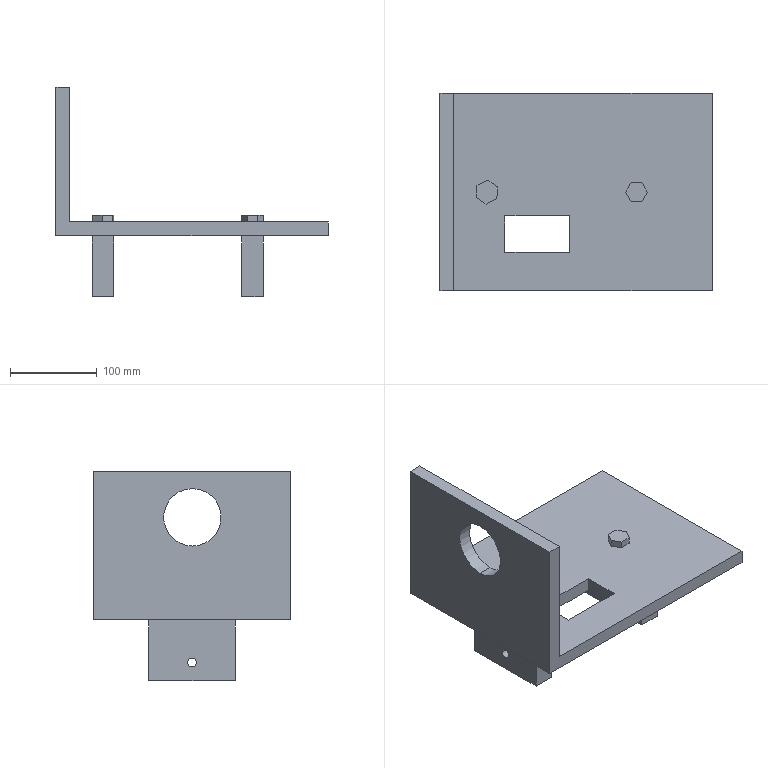Component | SolidWorks | SupportPlate2-1 | 1 solid | 50 faces | box 313 x 227 x 241 mm | volume 1944542 mm3 | plane 40 | cylinder 10 | commonest cylinder face diameters 10 x4 12 x4 66 x2
build123d program:
from build123d import *

# Parameters (mm, degrees)
BOSS_EXTRUDE1_DEPTH  = 227
SKETCH2_R            = 6
CUT_EXTRUDE1_2_DEPTH = 227
BOSS_EXTRUDE2_DEPTH  = 8
SKETCH4_W            = 100
SKETCH4_H            = 25
BOSS_EXTRUDE3_DEPTH  = 70
SKETCH5_R            = 5
CUT_EXTRUDE2_DEPTH   = 445.761
SKETCH6_W            = 41.929
SKETCH6_H            = 74.66
CUT_EXTRUDE3_DEPTH   = 412.071
SKETCH1_R            = 33
CUT_EXTRUDE1_DEPTH   = 17


with BuildPart() as part:
    # Sketch1_2 → Boss-Extrude1 (new body)
    with BuildSketch(Plane(origin=(0, 0, 0), x_dir=(0, 0, -1), z_dir=(1, 0, 0))):
        Polygon((213, 0), (58, 0), (58, -16), (229, -16), (229, 297), (213, 297), align=None)
    extrude(amount=BOSS_EXTRUDE1_DEPTH)

    # Sketch2 → Cut-Extrude1_2 (cut)
    with BuildSketch(Plane(origin=(0, 0, -229), x_dir=(-1, 0, 0), z_dir=(0, 0, -1))):
        with Locations(Location((-113.5, 210, 0), (0, 0, 90))):
            Circle(SKETCH2_R)
        with Locations(Location((-113.5, 38, 0), (0, 0, 90))):
            Circle(SKETCH2_R)
    extrude(amount=-CUT_EXTRUDE1_2_DEPTH, mode=Mode.SUBTRACT)

    # Sketch3 → Boss-Extrude2 (add)
    with BuildSketch(Plane.XY.offset(-213)):
        Polygon((113.5, 197.557), (124.276, 203.778), (124.276, 216.222), (113.5, 222.443), (102.724, 216.222), (102.724, 203.778), align=None)
        Polygon((119.5, 25.645), (127.199, 37.019), (121.199, 49.373), (107.5, 50.355), (99.801, 38.981), (105.801, 26.627), align=None)
    extrude(amount=BOSS_EXTRUDE2_DEPTH)

    # Sketch4 → Boss-Extrude3 (add)
    with BuildSketch(Plane(origin=(0, 0, -229), x_dir=(-1, 0, 0), z_dir=(0, 0, -1))):
        with Locations((-113.5, 210)):
            Rectangle(SKETCH4_W, SKETCH4_H)
        with Locations((-113.5, 38)):
            Rectangle(SKETCH4_W, SKETCH4_H)
    extrude(amount=BOSS_EXTRUDE3_DEPTH)

    # Sketch5 → Cut-Extrude2 (cut, through all)
    with BuildSketch(Plane(origin=(0, 222.5, 0), x_dir=(1, 0, 0), z_dir=(0, 1, 0))):
        with Locations(Location((113.5, 278, 0), (0, 0, 180))):
            Circle(SKETCH5_R)
    extrude(amount=-CUT_EXTRUDE2_DEPTH, mode=Mode.SUBTRACT)

    # Sketch6 → Cut-Extrude3 (cut, through all)
    with BuildSketch(Plane(origin=(0, 0, -229), x_dir=(-1, 0, 0), z_dir=(0, 0, -1))):
        with Locations((-161.854, 96)):
            Rectangle(SKETCH6_W, SKETCH6_H)
    extrude(amount=-CUT_EXTRUDE3_DEPTH, mode=Mode.SUBTRACT)

    # Sketch1 → Cut-Extrude1 (cut)
    with BuildSketch(Plane(origin=(0, 0, 0), x_dir=(1, 0, 0), z_dir=(0, 1, 0))):
        with Locations(Location((114, 111, 0), (0, 0, 270))):
            Circle(SKETCH1_R)
    extrude(amount=-CUT_EXTRUDE1_DEPTH, mode=Mode.SUBTRACT)


solid = part.part

# Placed as in the assembly
solid = solid.moved(Location((577.733, 129.31, 0.9999), (0, 0, -90)))